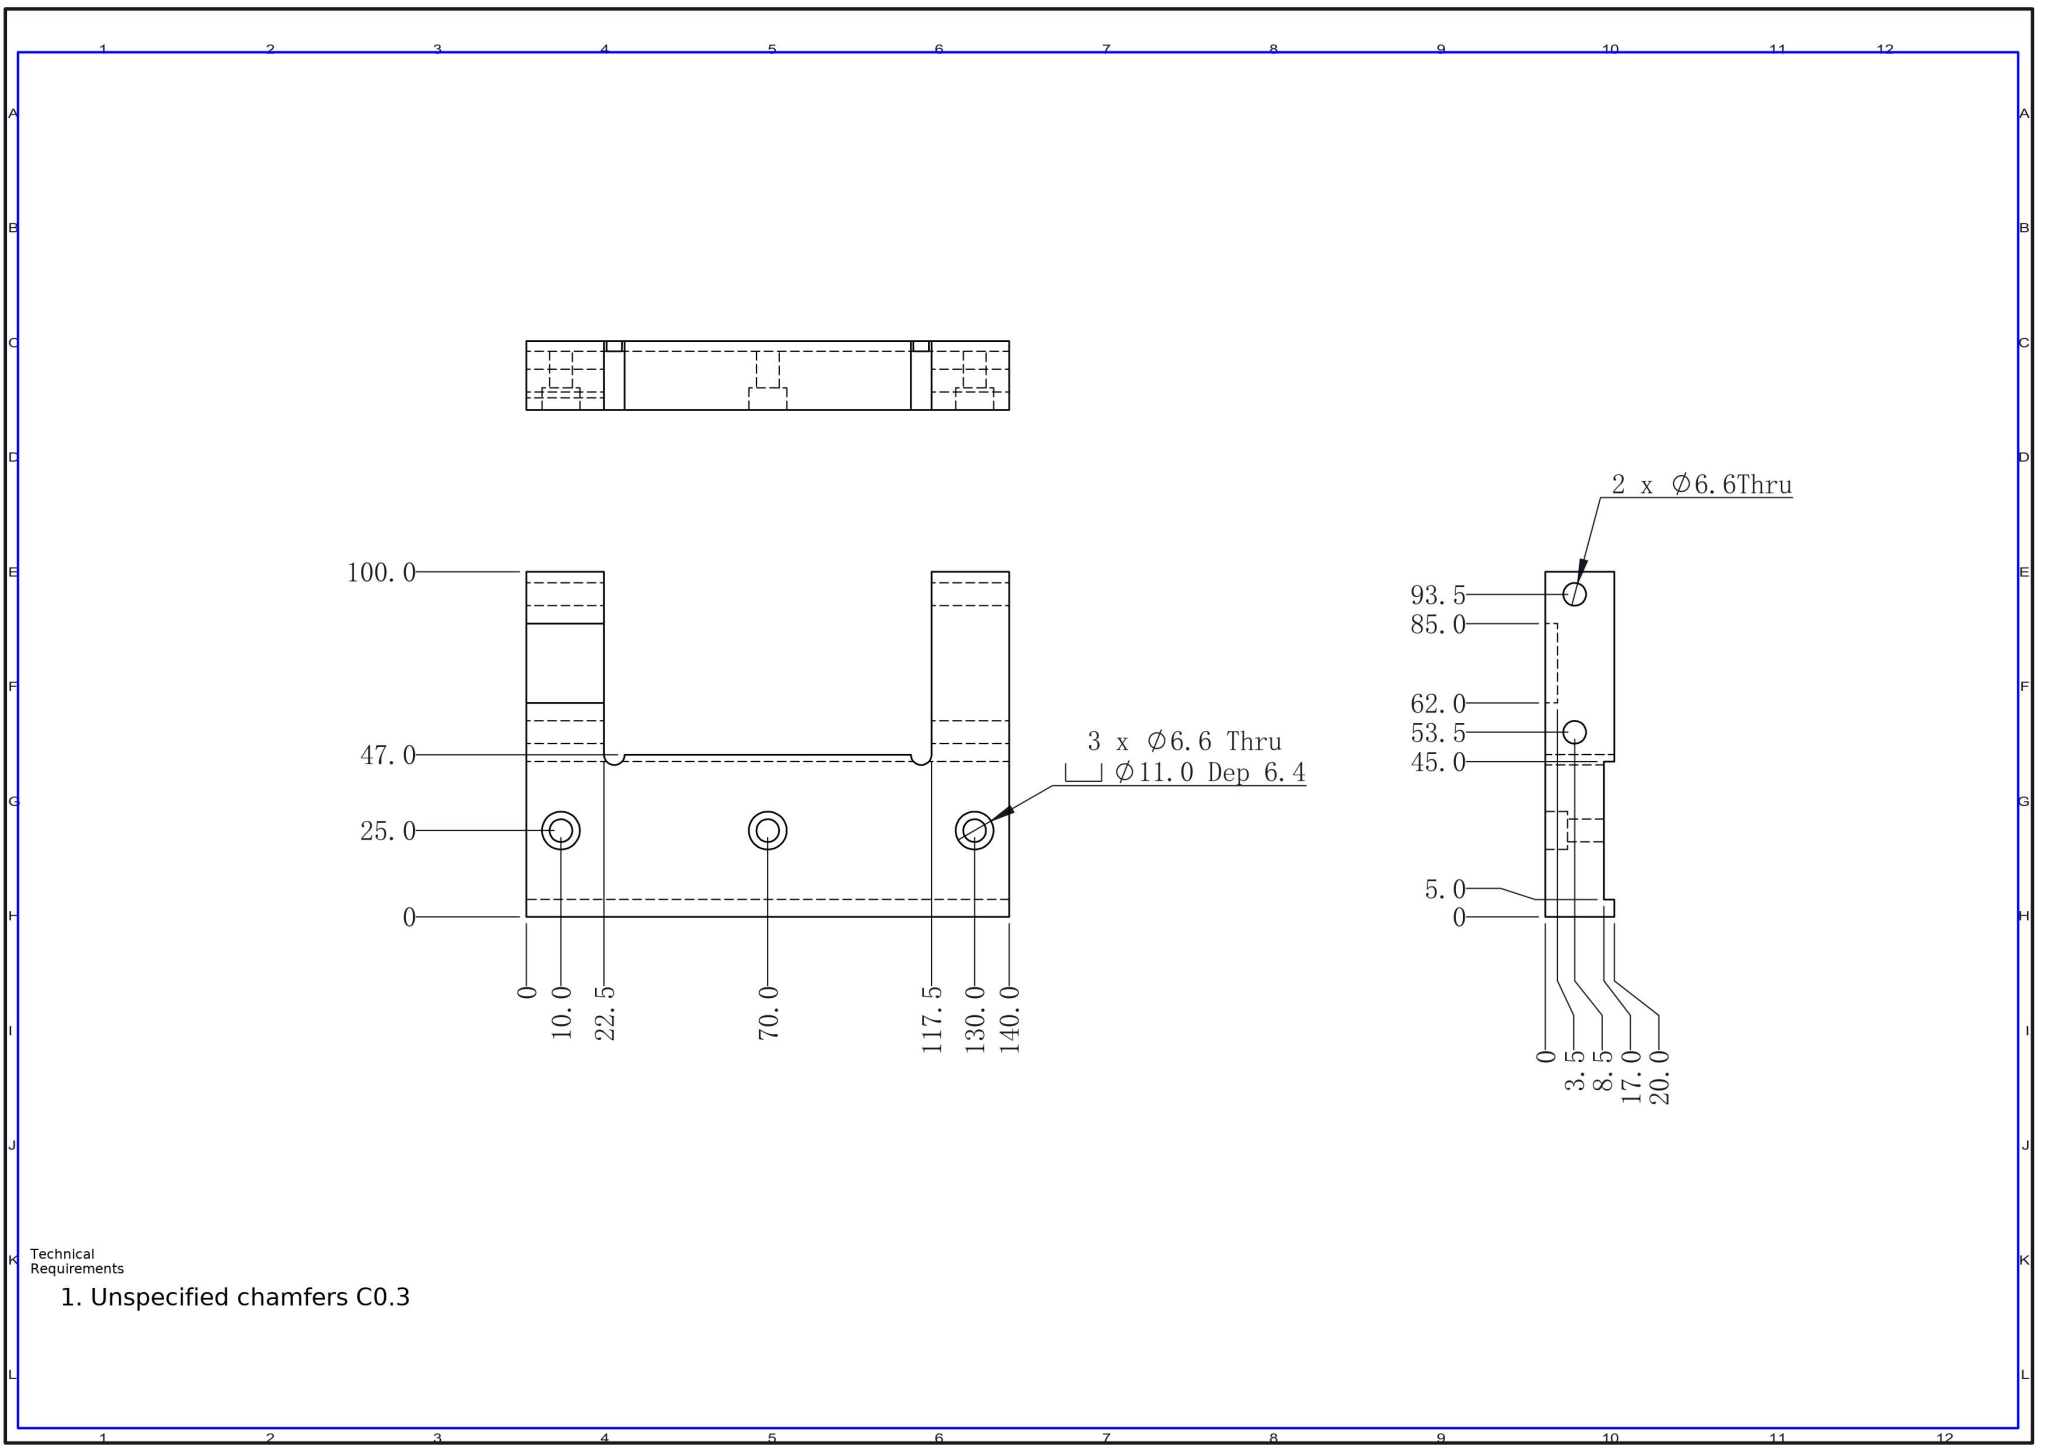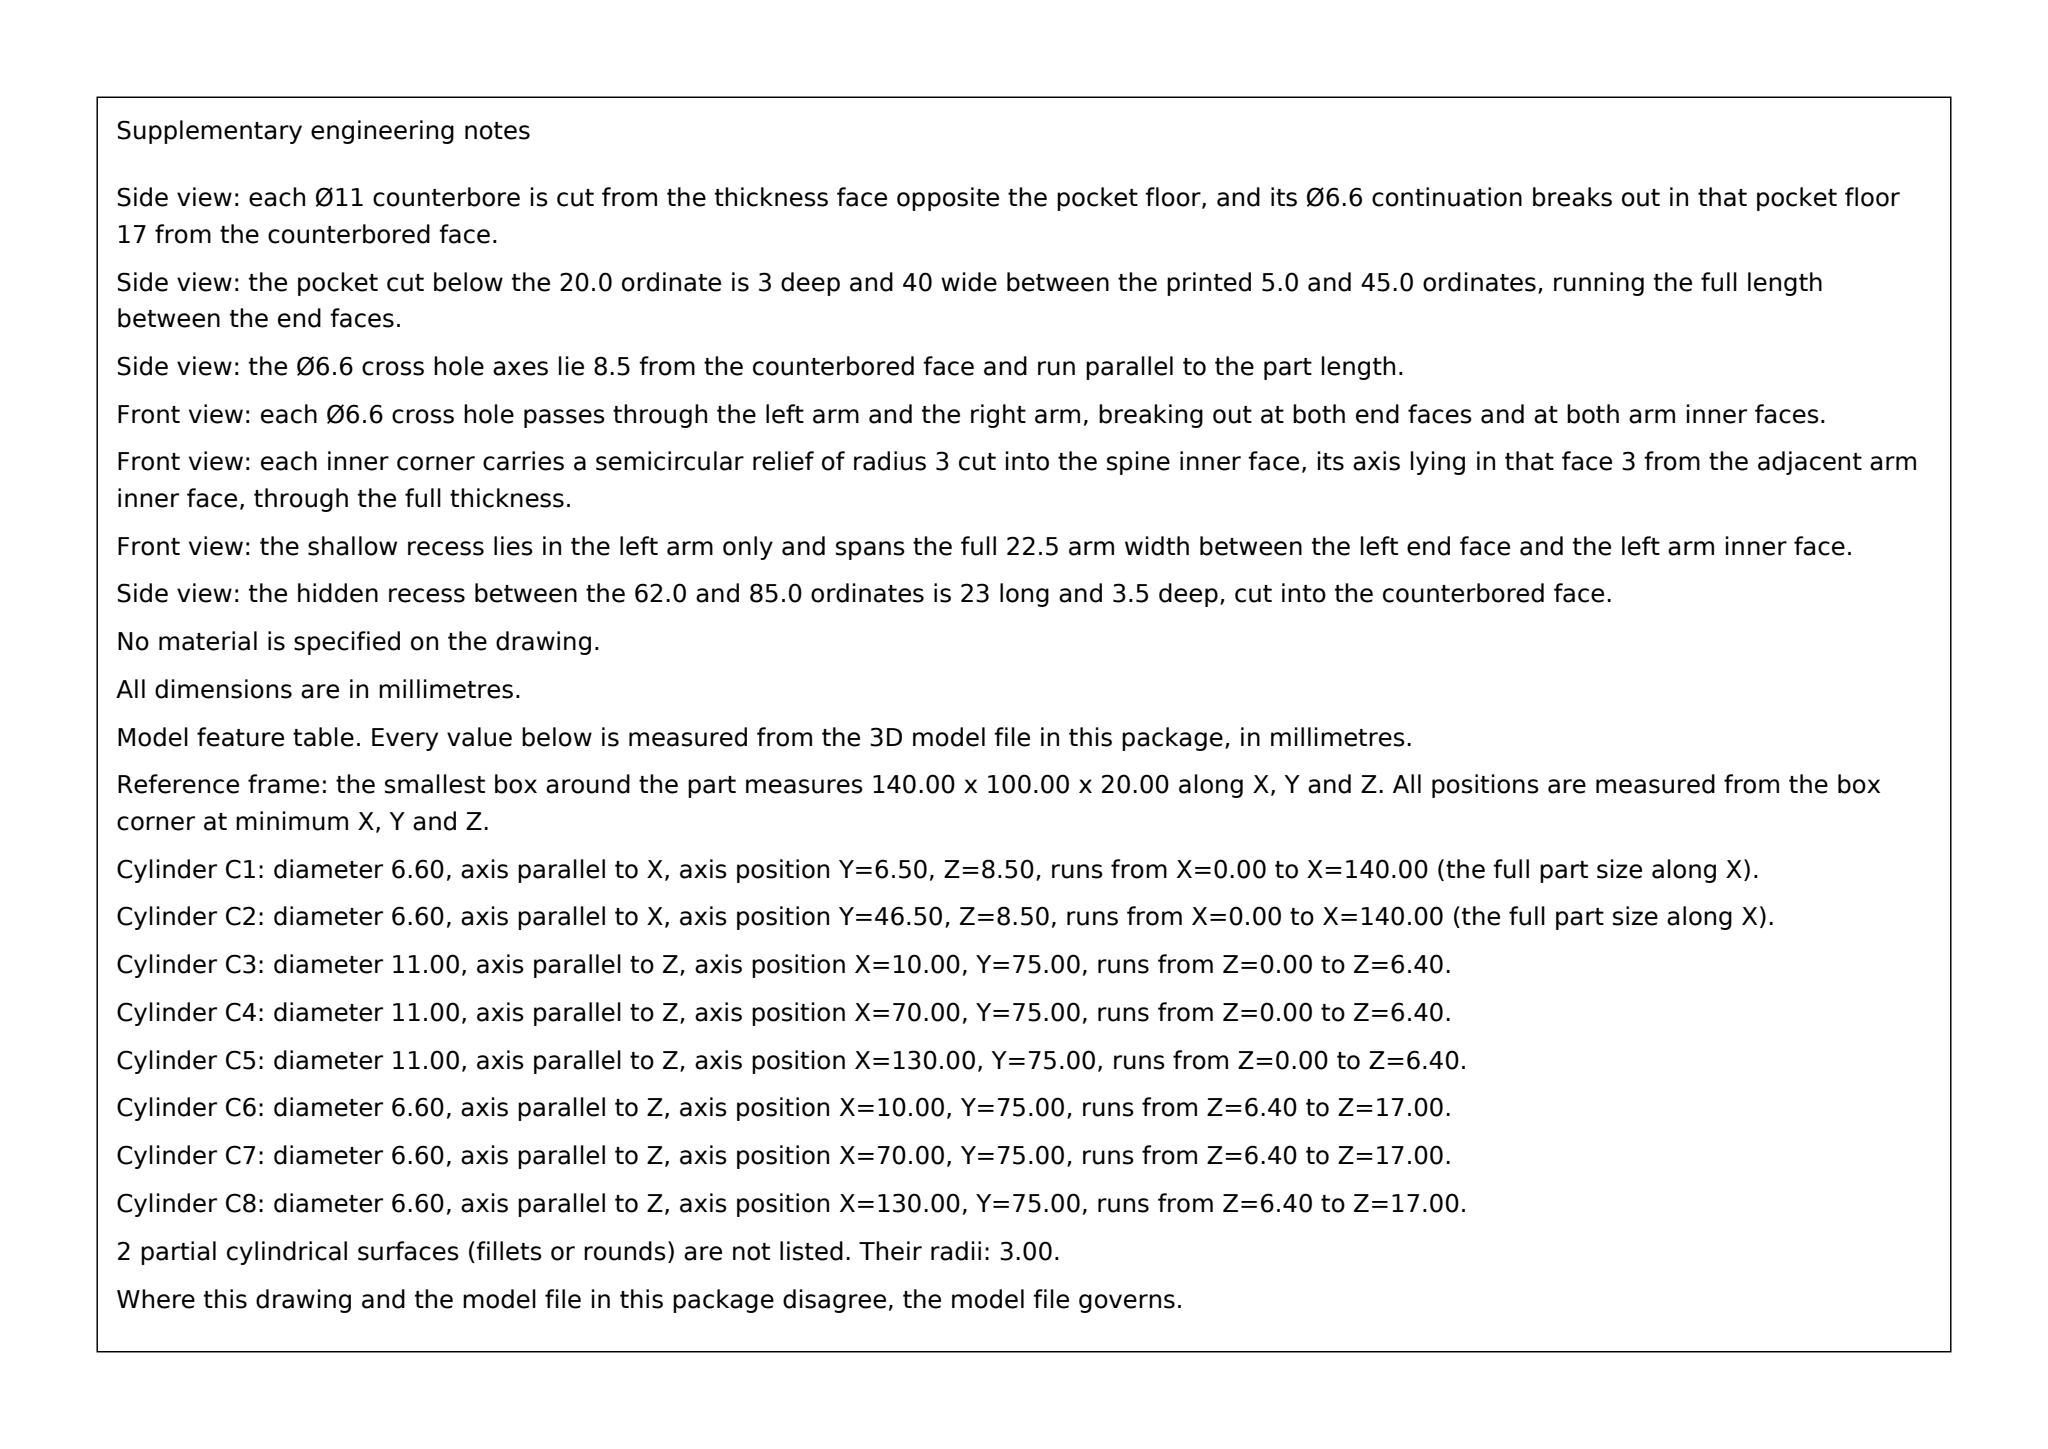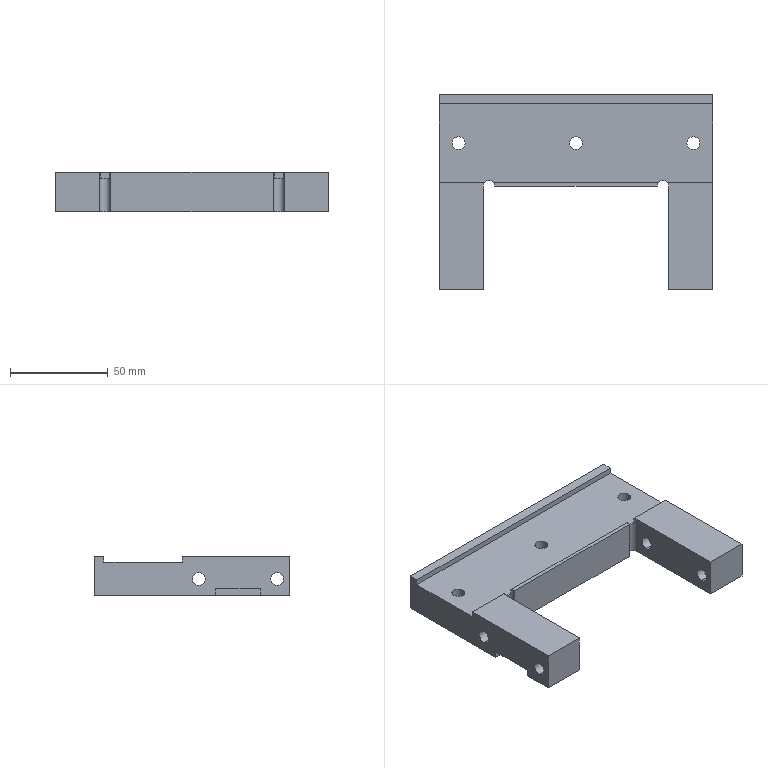Part | SolidWorks | mm | 1 solid | 47 faces | box 140 x 100 x 20 mm | volume 154150 mm3 | plane 25 | cylinder 22 | commonest cylinder face diameters 6.6 x14 11 x6 6 x2
Drawing notes:
4X Ø6.6 THRU ALONG X, 2 PER LEG (X 0-22.5 & 117.5-140), FULL 22.5 LEG THK | from the solid: cyl Ø6.6 axis x at (y6.5,z8.5) & (y46.5,z8.5), len 22.5, count 4; x-planes 0/22.5 & 117.5/140
FRONT FACE SLOT LEFT LEG 62.0-85.0, 3.5 DP, FULL 22.5 LEG WIDTH | from the solid: y planes 15 & 38 (=dwg 85.0 & 62.0) 1 each; z plane 3.5 count 1 = slot floor from front face z0
BACK RECESS BTWN LEGS X22.5-117.5, Y5.0-45.0, 3 DP FROM BACK FACE | from the solid: z plane 17.0 count 1 = floor 3 below back face z20; y planes 55 & 95 (=dwg 45.0 & 5.0); Ø6.6 thru len 10.6 = 17.0-6.4
build123d program:
from build123d import *

# Parameters (mm, degrees)
SKETCH1_W                                       = 140
SKETCH1_H                                       = 100
BOSS_EXTRUDE1_DEPTH                             = 20
SKETCH2_W                                       = 140
SKETCH2_H                                       = 40
CUT_EXTRUDE1_DEPTH                              = 3
M6_HEX_SOCKET_HEAD_CAP_SCREW_CBORE1_D           = 6.6
M6_HEX_SOCKET_HEAD_CAP_SCREW_CBORE1_CBORE_D     = 11
M6_HEX_SOCKET_HEAD_CAP_SCREW_CBORE1_CBORE_DEPTH = 6.4
SKETCH8_W                                       = 95
SKETCH8_H                                       = 53
CUT_EXTRUDE2_DEPTH                              = 174.205
M6_CLEARANCE_HOLE1_D                            = 6.6
CUT_EXTRUDE3_REACH                              = 175.205
SKETCH11_W                                      = 3.5
SKETCH11_H                                      = 23
SKETCH12_R                                      = 3
CUT_EXTRUDE4_DEPTH                              = 174.205


with BuildPart() as part:
    # Sketch1 → Boss-Extrude1 (new body)
    with BuildSketch(Plane.XY):
        with Locations((70, -50)):
            Rectangle(SKETCH1_W, SKETCH1_H)
    extrude(amount=BOSS_EXTRUDE1_DEPTH)

    # Sketch2 → Cut-Extrude1 (cut)
    with BuildSketch(Plane.XY.offset(20)):
        with Locations((70, -25)):
            Rectangle(SKETCH2_W, SKETCH2_H)
    extrude(amount=-CUT_EXTRUDE1_DEPTH, mode=Mode.SUBTRACT)

    # M6 Hex Socket Head Cap Screw CBORE1 (through all)
    with Locations(Plane(origin=(0, 0, 0), x_dir=(-1, 0, 0), z_dir=(0, 0, -1))):
        with Locations((-10, -25), (-70, -25), (-130, -25)):
            CounterBoreHole(M6_HEX_SOCKET_HEAD_CAP_SCREW_CBORE1_D / 2, M6_HEX_SOCKET_HEAD_CAP_SCREW_CBORE1_CBORE_D / 2, M6_HEX_SOCKET_HEAD_CAP_SCREW_CBORE1_CBORE_DEPTH)

    # Sketch8 → Cut-Extrude2 (cut, through all)
    with BuildSketch(Plane(origin=(0, 0, 0), x_dir=(-1, 0, 0), z_dir=(0, 0, -1))):
        with Locations((-70, -73.5)):
            Rectangle(SKETCH8_W, SKETCH8_H)
    extrude(amount=-CUT_EXTRUDE2_DEPTH, mode=Mode.SUBTRACT)

    # M6 Clearance Hole1 (through all)
    with Locations(Plane.ZY):
        with Locations((8.5, -53.5), (8.5, -93.5)):
            Hole(M6_CLEARANCE_HOLE1_D / 2)

    # Sketch11 → Cut-Extrude3 (cut, up to next)
    with BuildSketch(Plane.ZY, mode=Mode.PRIVATE) as cut_extrude3_sk1:
        with Locations((1.75, -73.5)):
            Rectangle(SKETCH11_W, SKETCH11_H)
    cut_extrude3_tool1 = extrude(cut_extrude3_sk1.sketch, amount=-CUT_EXTRUDE3_REACH, mode=Mode.PRIVATE) & part.part
    add(cut_extrude3_tool1.solids().sort_by_distance((0, -73.5, 1.75))[0], mode=Mode.SUBTRACT)

    # Sketch12 → Cut-Extrude4 (cut, through all)
    with BuildSketch(Plane(origin=(0, 0, 0), x_dir=(-1, 0, 0), z_dir=(0, 0, -1))):
        with Locations((-25.5, -47)):
            Circle(SKETCH12_R)
        with Locations((-114.5, -47)):
            Circle(SKETCH12_R)
    extrude(amount=-CUT_EXTRUDE4_DEPTH, mode=Mode.SUBTRACT)


solid = part.part